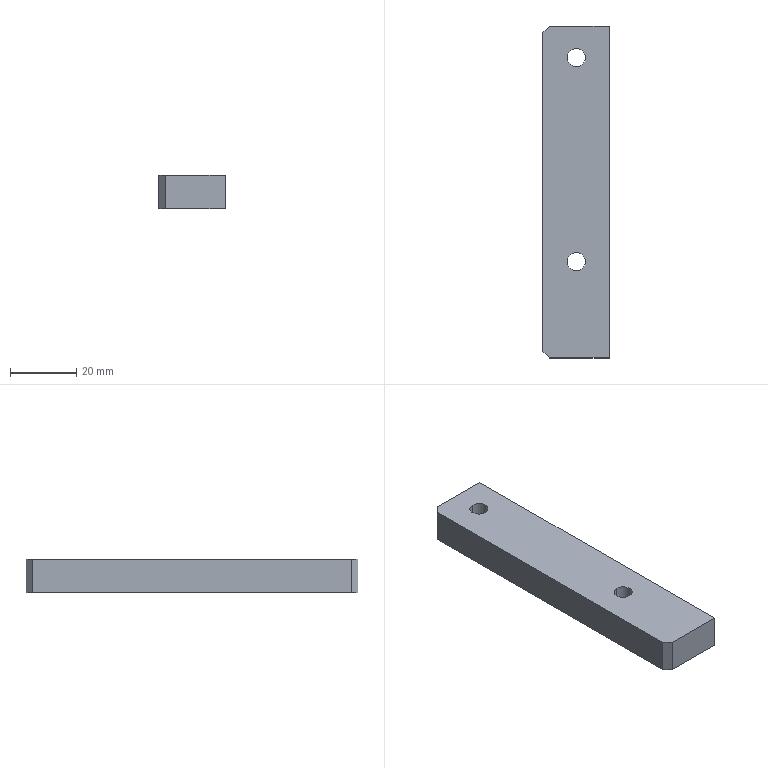Component | SolidWorks | BladeHolder-1 | 1 solid | 18 faces | box 20 x 100 x 10 mm | volume 18828 mm3 | plane 10 | cylinder 8 | commonest cylinder face diameters 12.238 x4 5.5 x4
build123d program:
from build123d import *

# Parameters (mm, degrees)
BOSS_EXTRUDE1_DEPTH                     = 10
M5_HEX_HEAD_BOLT_POST_HOLE1_D           = 5.5
M5_HEX_HEAD_BOLT_POST_HOLE1_CBORE_D     = 12.238
M5_HEX_HEAD_BOLT_POST_HOLE1_CBORE_DEPTH = 3.5


with BuildPart() as part:
    # Sketch1 → Boss-Extrude1 (new body)
    with BuildSketch(Plane.XY):
        Polygon((-48, 25), (-50, 23), (-50, 5), (50, 5), (50, 23), (48, 25), align=None)
    extrude(amount=BOSS_EXTRUDE1_DEPTH)

    # M5 Hex Head Bolt Post Hole1 (through all)
    with Locations(Plane.XY.offset(10)):
        with Locations((-40.5, 14.895), (21, 14.895)):
            CounterBoreHole(M5_HEX_HEAD_BOLT_POST_HOLE1_D / 2, M5_HEX_HEAD_BOLT_POST_HOLE1_CBORE_D / 2, M5_HEX_HEAD_BOLT_POST_HOLE1_CBORE_DEPTH)


solid = part.part

# Placed as in the assembly
solid = solid.moved(Location((-399.772, -298.766, 893.7), (180, 0, 90)))
STEP:
#1=COLOUR_RGB('',0.7922,0.8196,0.9333);
#2=FILL_AREA_STYLE_COLOUR('',#1);
#3=FILL_AREA_STYLE('',(#2));
#4=SURFACE_STYLE_FILL_AREA(#3);
#5=SURFACE_SIDE_STYLE('',(#4));
#6=SURFACE_STYLE_USAGE(.BOTH.,#5);
#7=PRESENTATION_STYLE_ASSIGNMENT((#6));
#8=CARTESIAN_POINT('',(-16.325,-9.927,34.929));
#9=VERTEX_POINT('',#8);
#10=CARTESIAN_POINT('',(-16.325,-10.409,34.929));
#11=VERTEX_POINT('',#10);
#12=CARTESIAN_POINT('',(-16.325,-10.168,34.929));
#13=DIRECTION('',(0.,0.,-1.));
#14=DIRECTION('',(0.,-1.,0.));
#15=AXIS2_PLACEMENT_3D('',#12,#13,#14);
#16=CIRCLE('',#15,0.2409);
#17=EDGE_CURVE('',#9,#11,#16,.T.);
#18=ORIENTED_EDGE('',*,*,#17,.F.);
#19=CARTESIAN_POINT('',(-16.325,-9.927,34.791));
#20=VERTEX_POINT('',#19);
#21=CARTESIAN_POINT('',(-16.325,-9.927,34.791));
#22=DIRECTION('',(0.,0.,-1.));
#23=VECTOR('',#22,39.37);
#24=LINE('',#21,#23);
#25=EDGE_CURVE('',#9,#20,#24,.T.);
#26=ORIENTED_EDGE('',*,*,#25,.T.);
#27=CARTESIAN_POINT('',(-16.325,-10.409,34.791));
#28=VERTEX_POINT('',#27);
#29=CARTESIAN_POINT('',(-16.325,-10.168,34.791));
#30=DIRECTION('',(0.,0.,-1.));
#31=DIRECTION('',(0.,-1.,0.));
#32=AXIS2_PLACEMENT_3D('',#29,#30,#31);
#33=CIRCLE('',#32,0.2409);
#34=EDGE_CURVE('',#20,#28,#33,.T.);
#35=ORIENTED_EDGE('',*,*,#34,.T.);
#36=CARTESIAN_POINT('',(-16.325,-10.409,34.791));
#37=DIRECTION('',(0.,0.,-1.));
#38=VECTOR('',#37,39.37);
#39=LINE('',#36,#38);
#40=EDGE_CURVE('',#11,#28,#39,.T.);
#41=ORIENTED_EDGE('',*,*,#40,.F.);
#42=EDGE_LOOP('',(#18,#26,#35,#41));
#43=FACE_OUTER_BOUND('',#42,.T.);
#44=CARTESIAN_POINT('',(-16.325,-10.168,34.791));
#45=DIRECTION('',(0.,0.,-1.));
#46=DIRECTION('',(0.,-1.,0.));
#47=AXIS2_PLACEMENT_3D('',#44,#45,#46);
#48=CYLINDRICAL_SURFACE('',#47,0.2409);
#49=ADVANCED_FACE('',(#43),#48,.F.);
#50=CARTESIAN_POINT('',(-16.325,-10.06,35.185));
#51=VERTEX_POINT('',#50);
#52=CARTESIAN_POINT('',(-16.325,-10.276,35.185));
#53=VERTEX_POINT('',#52);
#54=CARTESIAN_POINT('',(-16.325,-10.168,35.185));
#55=DIRECTION('',(0.,0.,-1.));
#56=DIRECTION('',(0.,-1.,0.));
#57=AXIS2_PLACEMENT_3D('',#54,#55,#56);
#58=CIRCLE('',#57,0.1083);
#59=EDGE_CURVE('',#51,#53,#58,.T.);
#60=ORIENTED_EDGE('',*,*,#59,.F.);
#61=CARTESIAN_POINT('',(-16.325,-10.06,34.929));
#62=VERTEX_POINT('',#61);
#63=CARTESIAN_POINT('',(-16.325,-10.06,34.791));
#64=DIRECTION('',(0.,0.,-1.));
#65=VECTOR('',#64,39.37);
#66=LINE('',#63,#65);
#67=EDGE_CURVE('',#51,#62,#66,.T.);
#68=ORIENTED_EDGE('',*,*,#67,.T.);
#69=CARTESIAN_POINT('',(-16.325,-10.276,34.929));
#70=VERTEX_POINT('',#69);
#71=CARTESIAN_POINT('',(-16.325,-10.168,34.929));
#72=DIRECTION('',(0.,0.,-1.));
#73=DIRECTION('',(0.,-1.,0.));
#74=AXIS2_PLACEMENT_3D('',#71,#72,#73);
#75=CIRCLE('',#74,0.1083);
#76=EDGE_CURVE('',#62,#70,#75,.T.);
#77=ORIENTED_EDGE('',*,*,#76,.T.);
#78=CARTESIAN_POINT('',(-16.325,-10.276,34.791));
#79=DIRECTION('',(0.,0.,-1.));
#80=VECTOR('',#79,39.37);
#81=LINE('',#78,#80);
#82=EDGE_CURVE('',#53,#70,#81,.T.);
#83=ORIENTED_EDGE('',*,*,#82,.F.);
#84=EDGE_LOOP('',(#60,#68,#77,#83));
#85=FACE_OUTER_BOUND('',#84,.T.);
#86=CARTESIAN_POINT('',(-16.325,-10.168,34.791));
#87=DIRECTION('',(0.,0.,-1.));
#88=DIRECTION('',(0.,-1.,0.));
#89=AXIS2_PLACEMENT_3D('',#86,#87,#88);
#90=CYLINDRICAL_SURFACE('',#89,0.1083);
#91=ADVANCED_FACE('',(#85),#90,.F.);
#92=CARTESIAN_POINT('',(-16.325,-12.348,34.929));
#93=VERTEX_POINT('',#92);
#94=CARTESIAN_POINT('',(-16.325,-12.83,34.929));
#95=VERTEX_POINT('',#94);
#96=CARTESIAN_POINT('',(-16.325,-12.589,34.929));
#97=DIRECTION('',(0.,0.,-1.));
#98=DIRECTION('',(0.,-1.,0.));
#99=AXIS2_PLACEMENT_3D('',#96,#97,#98);
#100=CIRCLE('',#99,0.2409);
#101=EDGE_CURVE('',#93,#95,#100,.T.);
#102=ORIENTED_EDGE('',*,*,#101,.F.);
#103=CARTESIAN_POINT('',(-16.325,-12.348,34.791));
#104=VERTEX_POINT('',#103);
#105=CARTESIAN_POINT('',(-16.325,-12.348,34.791));
#106=DIRECTION('',(0.,0.,-1.));
#107=VECTOR('',#106,39.37);
#108=LINE('',#105,#107);
#109=EDGE_CURVE('',#93,#104,#108,.T.);
#110=ORIENTED_EDGE('',*,*,#109,.T.);
#111=CARTESIAN_POINT('',(-16.325,-12.83,34.791));
#112=VERTEX_POINT('',#111);
#113=CARTESIAN_POINT('',(-16.325,-12.589,34.791));
#114=DIRECTION('',(0.,0.,-1.));
#115=DIRECTION('',(0.,-1.,0.));
#116=AXIS2_PLACEMENT_3D('',#113,#114,#115);
#117=CIRCLE('',#116,0.2409);
#118=EDGE_CURVE('',#104,#112,#117,.T.);
#119=ORIENTED_EDGE('',*,*,#118,.T.);
#120=CARTESIAN_POINT('',(-16.325,-12.83,34.791));
#121=DIRECTION('',(0.,0.,-1.));
#122=VECTOR('',#121,39.37);
#123=LINE('',#120,#122);
#124=EDGE_CURVE('',#95,#112,#123,.T.);
#125=ORIENTED_EDGE('',*,*,#124,.F.);
#126=EDGE_LOOP('',(#102,#110,#119,#125));
#127=FACE_OUTER_BOUND('',#126,.T.);
#128=CARTESIAN_POINT('',(-16.325,-12.589,34.791));
#129=DIRECTION('',(0.,0.,-1.));
#130=DIRECTION('',(0.,-1.,0.));
#131=AXIS2_PLACEMENT_3D('',#128,#129,#130);
#132=CYLINDRICAL_SURFACE('',#131,0.2409);
#133=ADVANCED_FACE('',(#127),#132,.F.);
#134=CARTESIAN_POINT('',(-16.325,-12.481,35.185));
#135=VERTEX_POINT('',#134);
#136=CARTESIAN_POINT('',(-16.325,-12.697,35.185));
#137=VERTEX_POINT('',#136);
#138=CARTESIAN_POINT('',(-16.325,-12.589,35.185));
#139=DIRECTION('',(0.,0.,-1.));
#140=DIRECTION('',(0.,-1.,0.));
#141=AXIS2_PLACEMENT_3D('',#138,#139,#140);
#142=CIRCLE('',#141,0.1083);
#143=EDGE_CURVE('',#135,#137,#142,.T.);
#144=ORIENTED_EDGE('',*,*,#143,.F.);
#145=CARTESIAN_POINT('',(-16.325,-12.481,34.929));
#146=VERTEX_POINT('',#145);
#147=CARTESIAN_POINT('',(-16.325,-12.481,34.791));
#148=DIRECTION('',(0.,0.,-1.));
#149=VECTOR('',#148,39.37);
#150=LINE('',#147,#149);
#151=EDGE_CURVE('',#135,#146,#150,.T.);
#152=ORIENTED_EDGE('',*,*,#151,.T.);
#153=CARTESIAN_POINT('',(-16.325,-12.697,34.929));
#154=VERTEX_POINT('',#153);
#155=CARTESIAN_POINT('',(-16.325,-12.589,34.929));
#156=DIRECTION('',(0.,0.,-1.));
#157=DIRECTION('',(0.,-1.,0.));
#158=AXIS2_PLACEMENT_3D('',#155,#156,#157);
#159=CIRCLE('',#158,0.1083);
#160=EDGE_CURVE('',#146,#154,#159,.T.);
#161=ORIENTED_EDGE('',*,*,#160,.T.);
#162=CARTESIAN_POINT('',(-16.325,-12.697,34.791));
#163=DIRECTION('',(0.,0.,-1.));
#164=VECTOR('',#163,39.37);
#165=LINE('',#162,#164);
#166=EDGE_CURVE('',#137,#154,#165,.T.);
#167=ORIENTED_EDGE('',*,*,#166,.F.);
#168=EDGE_LOOP('',(#144,#152,#161,#167));
#169=FACE_OUTER_BOUND('',#168,.T.);
#170=CARTESIAN_POINT('',(-16.325,-12.589,34.791));
#171=DIRECTION('',(0.,0.,-1.));
#172=DIRECTION('',(0.,-1.,0.));
#173=AXIS2_PLACEMENT_3D('',#170,#171,#172);
#174=CYLINDRICAL_SURFACE('',#173,0.1083);
#175=ADVANCED_FACE('',(#169),#174,.F.);
#176=CARTESIAN_POINT('',(-15.936,-13.731,35.185));
#177=VERTEX_POINT('',#176);
#178=CARTESIAN_POINT('',(-16.645,-13.731,35.185));
#179=VERTEX_POINT('',#178);
#180=CARTESIAN_POINT('',(-16.645,-13.731,35.185));
#181=DIRECTION('',(-1.,-0.,-0.));
#182=VECTOR('',#181,39.37);
#183=LINE('',#180,#182);
#184=EDGE_CURVE('',#177,#179,#183,.T.);
#185=ORIENTED_EDGE('',*,*,#184,.T.);
#186=CARTESIAN_POINT('',(-16.645,-13.731,34.791));
#187=VERTEX_POINT('',#186);
#188=CARTESIAN_POINT('',(-16.645,-13.731,34.791));
#189=DIRECTION('',(-0.,-0.,1.));
#190=VECTOR('',#189,39.37);
#191=LINE('',#188,#190);
#192=EDGE_CURVE('',#187,#179,#191,.T.);
#193=ORIENTED_EDGE('',*,*,#192,.F.);
#194=CARTESIAN_POINT('',(-15.936,-13.731,34.791));
#195=VERTEX_POINT('',#194);
#196=CARTESIAN_POINT('',(-16.645,-13.731,34.791));
#197=DIRECTION('',(-1.,-0.,-0.));
#198=VECTOR('',#197,39.37);
#199=LINE('',#196,#198);
#200=EDGE_CURVE('',#195,#187,#199,.T.);
#201=ORIENTED_EDGE('',*,*,#200,.F.);
#202=CARTESIAN_POINT('',(-15.936,-13.731,34.791));
#203=DIRECTION('',(-0.,-0.,1.));
#204=VECTOR('',#203,39.37);
#205=LINE('',#202,#204);
#206=EDGE_CURVE('',#195,#177,#205,.T.);
#207=ORIENTED_EDGE('',*,*,#206,.T.);
#208=EDGE_LOOP('',(#185,#193,#201,#207));
#209=FACE_OUTER_BOUND('',#208,.T.);
#210=CARTESIAN_POINT('',(-16.645,-13.731,34.791));
#211=DIRECTION('',(-0.,1.,0.));
#212=DIRECTION('',(0.,0.,-1.));
#213=AXIS2_PLACEMENT_3D('',#210,#211,#212);
#214=PLANE('',#213);
#215=ADVANCED_FACE('',(#209),#214,.F.);
#216=CARTESIAN_POINT('',(-16.723,-13.652,35.185));
#217=VERTEX_POINT('',#216);
#218=CARTESIAN_POINT('',(-16.723,-13.652,35.185));
#219=DIRECTION('',(-0.7071,0.7071,0.));
#220=VECTOR('',#219,39.37);
#221=LINE('',#218,#220);
#222=EDGE_CURVE('',#179,#217,#221,.T.);
#223=ORIENTED_EDGE('',*,*,#222,.T.);
#224=CARTESIAN_POINT('',(-16.723,-13.652,34.791));
#225=VERTEX_POINT('',#224);
#226=CARTESIAN_POINT('',(-16.723,-13.652,34.791));
#227=DIRECTION('',(-0.,-0.,1.));
#228=VECTOR('',#227,39.37);
#229=LINE('',#226,#228);
#230=EDGE_CURVE('',#225,#217,#229,.T.);
#231=ORIENTED_EDGE('',*,*,#230,.F.);
#232=CARTESIAN_POINT('',(-16.723,-13.652,34.791));
#233=DIRECTION('',(-0.7071,0.7071,0.));
#234=VECTOR('',#233,39.37);
#235=LINE('',#232,#234);
#236=EDGE_CURVE('',#187,#225,#235,.T.);
#237=ORIENTED_EDGE('',*,*,#236,.F.);
#238=ORIENTED_EDGE('',*,*,#192,.T.);
#239=EDGE_LOOP('',(#223,#231,#237,#238));
#240=FACE_OUTER_BOUND('',#239,.T.);
#241=CARTESIAN_POINT('',(-16.723,-13.652,34.791));
#242=DIRECTION('',(0.7071,0.7071,0.));
#243=DIRECTION('',(0.7071,-0.7071,-0.));
#244=AXIS2_PLACEMENT_3D('',#241,#242,#243);
#245=PLANE('',#244);
#246=ADVANCED_FACE('',(#240),#245,.F.);
#247=CARTESIAN_POINT('',(-16.723,-9.873,35.185));
#248=VERTEX_POINT('',#247);
#249=CARTESIAN_POINT('',(-16.723,-9.873,35.185));
#250=DIRECTION('',(-0.,1.,0.));
#251=VECTOR('',#250,39.37);
#252=LINE('',#249,#251);
#253=EDGE_CURVE('',#217,#248,#252,.T.);
#254=ORIENTED_EDGE('',*,*,#253,.T.);
#255=CARTESIAN_POINT('',(-16.723,-9.873,34.791));
#256=VERTEX_POINT('',#255);
#257=CARTESIAN_POINT('',(-16.723,-9.873,34.791));
#258=DIRECTION('',(-0.,-0.,1.));
#259=VECTOR('',#258,39.37);
#260=LINE('',#257,#259);
#261=EDGE_CURVE('',#256,#248,#260,.T.);
#262=ORIENTED_EDGE('',*,*,#261,.F.);
#263=CARTESIAN_POINT('',(-16.723,-9.873,34.791));
#264=DIRECTION('',(-0.,1.,0.));
#265=VECTOR('',#264,39.37);
#266=LINE('',#263,#265);
#267=EDGE_CURVE('',#225,#256,#266,.T.);
#268=ORIENTED_EDGE('',*,*,#267,.F.);
#269=ORIENTED_EDGE('',*,*,#230,.T.);
#270=EDGE_LOOP('',(#254,#262,#268,#269));
#271=FACE_OUTER_BOUND('',#270,.T.);
#272=CARTESIAN_POINT('',(-16.723,-9.873,34.791));
#273=DIRECTION('',(1.,0.,0.));
#274=DIRECTION('',(-0.,-0.,1.));
#275=AXIS2_PLACEMENT_3D('',#272,#273,#274);
#276=PLANE('',#275);
#277=ADVANCED_FACE('',(#271),#276,.F.);
#278=CARTESIAN_POINT('',(-16.645,-9.794,35.185));
#279=VERTEX_POINT('',#278);
#280=CARTESIAN_POINT('',(-16.723,-9.873,35.185));
#281=DIRECTION('',(0.7071,0.7071,0.));
#282=VECTOR('',#281,39.37);
#283=LINE('',#280,#282);
#284=EDGE_CURVE('',#248,#279,#283,.T.);
#285=ORIENTED_EDGE('',*,*,#284,.T.);
#286=CARTESIAN_POINT('',(-16.645,-9.794,34.791));
#287=VERTEX_POINT('',#286);
#288=CARTESIAN_POINT('',(-16.645,-9.794,34.791));
#289=DIRECTION('',(-0.,-0.,1.));
#290=VECTOR('',#289,39.37);
#291=LINE('',#288,#290);
#292=EDGE_CURVE('',#287,#279,#291,.T.);
#293=ORIENTED_EDGE('',*,*,#292,.F.);
#294=CARTESIAN_POINT('',(-16.723,-9.873,34.791));
#295=DIRECTION('',(0.7071,0.7071,0.));
#296=VECTOR('',#295,39.37);
#297=LINE('',#294,#296);
#298=EDGE_CURVE('',#256,#287,#297,.T.);
#299=ORIENTED_EDGE('',*,*,#298,.F.);
#300=ORIENTED_EDGE('',*,*,#261,.T.);
#301=EDGE_LOOP('',(#285,#293,#299,#300));
#302=FACE_OUTER_BOUND('',#301,.T.);
#303=CARTESIAN_POINT('',(-16.723,-9.873,34.791));
#304=DIRECTION('',(0.7071,-0.7071,-0.));
#305=DIRECTION('',(-0.7071,-0.7071,-0.));
#306=AXIS2_PLACEMENT_3D('',#303,#304,#305);
#307=PLANE('',#306);
#308=ADVANCED_FACE('',(#302),#307,.F.);
#309=CARTESIAN_POINT('',(-15.936,-9.794,35.185));
#310=VERTEX_POINT('',#309);
#311=CARTESIAN_POINT('',(-16.645,-9.794,35.185));
#312=DIRECTION('',(1.,0.,0.));
#313=VECTOR('',#312,39.37);
#314=LINE('',#311,#313);
#315=EDGE_CURVE('',#279,#310,#314,.T.);
#316=ORIENTED_EDGE('',*,*,#315,.T.);
#317=CARTESIAN_POINT('',(-15.936,-9.794,34.791));
#318=VERTEX_POINT('',#317);
#319=CARTESIAN_POINT('',(-15.936,-9.794,34.791));
#320=DIRECTION('',(-0.,-0.,1.));
#321=VECTOR('',#320,39.37);
#322=LINE('',#319,#321);
#323=EDGE_CURVE('',#318,#310,#322,.T.);
#324=ORIENTED_EDGE('',*,*,#323,.F.);
#325=CARTESIAN_POINT('',(-16.645,-9.794,34.791));
#326=DIRECTION('',(1.,0.,0.));
#327=VECTOR('',#326,39.37);
#328=LINE('',#325,#327);
#329=EDGE_CURVE('',#287,#318,#328,.T.);
#330=ORIENTED_EDGE('',*,*,#329,.F.);
#331=ORIENTED_EDGE('',*,*,#292,.T.);
#332=EDGE_LOOP('',(#316,#324,#330,#331));
#333=FACE_OUTER_BOUND('',#332,.T.);
#334=CARTESIAN_POINT('',(-16.645,-9.794,34.791));
#335=DIRECTION('',(0.,-1.,-0.));
#336=DIRECTION('',(-0.,-0.,1.));
#337=AXIS2_PLACEMENT_3D('',#334,#335,#336);
#338=PLANE('',#337);
#339=ADVANCED_FACE('',(#333),#338,.F.);
#340=CARTESIAN_POINT('',(-15.936,-9.794,35.185));
#341=DIRECTION('',(0.,-1.,-0.));
#342=VECTOR('',#341,39.37);
#343=LINE('',#340,#342);
#344=EDGE_CURVE('',#310,#177,#343,.T.);
#345=ORIENTED_EDGE('',*,*,#344,.T.);
#346=ORIENTED_EDGE('',*,*,#206,.F.);
#347=CARTESIAN_POINT('',(-15.936,-9.794,34.791));
#348=DIRECTION('',(0.,-1.,-0.));
#349=VECTOR('',#348,39.37);
#350=LINE('',#347,#349);
#351=EDGE_CURVE('',#318,#195,#350,.T.);
#352=ORIENTED_EDGE('',*,*,#351,.F.);
#353=ORIENTED_EDGE('',*,*,#323,.T.);
#354=EDGE_LOOP('',(#345,#346,#352,#353));
#355=FACE_OUTER_BOUND('',#354,.T.);
#356=CARTESIAN_POINT('',(-15.936,-9.794,34.791));
#357=DIRECTION('',(-1.,-0.,-0.));
#358=DIRECTION('',(0.,0.,-1.));
#359=AXIS2_PLACEMENT_3D('',#356,#357,#358);
#360=PLANE('',#359);
#361=ADVANCED_FACE('',(#355),#360,.F.);
#362=CARTESIAN_POINT('',(-16.325,-10.168,34.791));
#363=DIRECTION('',(0.,0.,-1.));
#364=DIRECTION('',(0.,-1.,0.));
#365=AXIS2_PLACEMENT_3D('',#362,#363,#364);
#366=CIRCLE('',#365,0.2409);
#367=EDGE_CURVE('',#28,#20,#366,.T.);
#368=ORIENTED_EDGE('',*,*,#367,.F.);
#369=ORIENTED_EDGE('',*,*,#34,.F.);
#370=EDGE_LOOP('',(#368,#369));
#371=FACE_BOUND('',#370,.T.);
#372=CARTESIAN_POINT('',(-16.325,-12.589,34.791));
#373=DIRECTION('',(0.,0.,-1.));
#374=DIRECTION('',(0.,-1.,0.));
#375=AXIS2_PLACEMENT_3D('',#372,#373,#374);
#376=CIRCLE('',#375,0.2409);
#377=EDGE_CURVE('',#112,#104,#376,.T.);
#378=ORIENTED_EDGE('',*,*,#377,.F.);
#379=ORIENTED_EDGE('',*,*,#118,.F.);
#380=EDGE_LOOP('',(#378,#379));
#381=FACE_BOUND('',#380,.T.);
#382=ORIENTED_EDGE('',*,*,#200,.T.);
#383=ORIENTED_EDGE('',*,*,#236,.T.);
#384=ORIENTED_EDGE('',*,*,#267,.T.);
#385=ORIENTED_EDGE('',*,*,#298,.T.);
#386=ORIENTED_EDGE('',*,*,#329,.T.);
#387=ORIENTED_EDGE('',*,*,#351,.T.);
#388=EDGE_LOOP('',(#382,#383,#384,#385,#386,#387));
#389=FACE_OUTER_BOUND('',#388,.T.);
#390=CARTESIAN_POINT('',(-15.739,-11.762,34.791));
#391=DIRECTION('',(0.,0.,-1.));
#392=DIRECTION('',(0.,-1.,-0.));
#393=AXIS2_PLACEMENT_3D('',#390,#391,#392);
#394=PLANE('',#393);
#395=ADVANCED_FACE('',(#371,#381,#389),#394,.T.);
#396=CARTESIAN_POINT('',(-16.325,-10.168,35.185));
#397=DIRECTION('',(0.,0.,-1.));
#398=DIRECTION('',(0.,-1.,0.));
#399=AXIS2_PLACEMENT_3D('',#396,#397,#398);
#400=CIRCLE('',#399,0.1083);
#401=EDGE_CURVE('',#53,#51,#400,.T.);
#402=ORIENTED_EDGE('',*,*,#401,.T.);
#403=ORIENTED_EDGE('',*,*,#59,.T.);
#404=EDGE_LOOP('',(#402,#403));
#405=FACE_BOUND('',#404,.T.);
#406=CARTESIAN_POINT('',(-16.325,-12.589,35.185));
#407=DIRECTION('',(0.,0.,-1.));
#408=DIRECTION('',(0.,-1.,0.));
#409=AXIS2_PLACEMENT_3D('',#406,#407,#408);
#410=CIRCLE('',#409,0.1083);
#411=EDGE_CURVE('',#137,#135,#410,.T.);
#412=ORIENTED_EDGE('',*,*,#411,.T.);
#413=ORIENTED_EDGE('',*,*,#143,.T.);
#414=EDGE_LOOP('',(#412,#413));
#415=FACE_BOUND('',#414,.T.);
#416=ORIENTED_EDGE('',*,*,#184,.F.);
#417=ORIENTED_EDGE('',*,*,#344,.F.);
#418=ORIENTED_EDGE('',*,*,#315,.F.);
#419=ORIENTED_EDGE('',*,*,#284,.F.);
#420=ORIENTED_EDGE('',*,*,#253,.F.);
#421=ORIENTED_EDGE('',*,*,#222,.F.);
#422=EDGE_LOOP('',(#416,#417,#418,#419,#420,#421));
#423=FACE_OUTER_BOUND('',#422,.T.);
#424=CARTESIAN_POINT('',(-15.739,-11.762,35.185));
#425=DIRECTION('',(0.,0.,-1.));
#426=DIRECTION('',(0.,-1.,-0.));
#427=AXIS2_PLACEMENT_3D('',#424,#425,#426);
#428=PLANE('',#427);
#429=ADVANCED_FACE('',(#405,#415,#423),#428,.F.);
#430=ORIENTED_EDGE('',*,*,#151,.F.);
#431=ORIENTED_EDGE('',*,*,#411,.F.);
#432=ORIENTED_EDGE('',*,*,#166,.T.);
#433=CARTESIAN_POINT('',(-16.325,-12.589,34.929));
#434=DIRECTION('',(0.,0.,-1.));
#435=DIRECTION('',(0.,-1.,0.));
#436=AXIS2_PLACEMENT_3D('',#433,#434,#435);
#437=CIRCLE('',#436,0.1083);
#438=EDGE_CURVE('',#154,#146,#437,.T.);
#439=ORIENTED_EDGE('',*,*,#438,.T.);
#440=EDGE_LOOP('',(#430,#431,#432,#439));
#441=FACE_OUTER_BOUND('',#440,.T.);
#442=CARTESIAN_POINT('',(-16.325,-12.589,34.791));
#443=DIRECTION('',(0.,0.,-1.));
#444=DIRECTION('',(0.,-1.,0.));
#445=AXIS2_PLACEMENT_3D('',#442,#443,#444);
#446=CYLINDRICAL_SURFACE('',#445,0.1083);
#447=ADVANCED_FACE('',(#441),#446,.F.);
#448=ORIENTED_EDGE('',*,*,#438,.F.);
#449=ORIENTED_EDGE('',*,*,#160,.F.);
#450=EDGE_LOOP('',(#448,#449));
#451=FACE_BOUND('',#450,.T.);
#452=CARTESIAN_POINT('',(-16.325,-12.589,34.929));
#453=DIRECTION('',(0.,0.,-1.));
#454=DIRECTION('',(0.,-1.,0.));
#455=AXIS2_PLACEMENT_3D('',#452,#453,#454);
#456=CIRCLE('',#455,0.2409);
#457=EDGE_CURVE('',#95,#93,#456,.T.);
#458=ORIENTED_EDGE('',*,*,#457,.T.);
#459=ORIENTED_EDGE('',*,*,#101,.T.);
#460=EDGE_LOOP('',(#458,#459));
#461=FACE_OUTER_BOUND('',#460,.T.);
#462=CARTESIAN_POINT('',(-16.325,-12.697,34.929));
#463=DIRECTION('',(-0.,-0.,1.));
#464=DIRECTION('',(-0.,1.,0.));
#465=AXIS2_PLACEMENT_3D('',#462,#463,#464);
#466=PLANE('',#465);
#467=ADVANCED_FACE('',(#451,#461),#466,.F.);
#468=ORIENTED_EDGE('',*,*,#109,.F.);
#469=ORIENTED_EDGE('',*,*,#457,.F.);
#470=ORIENTED_EDGE('',*,*,#124,.T.);
#471=ORIENTED_EDGE('',*,*,#377,.T.);
#472=EDGE_LOOP('',(#468,#469,#470,#471));
#473=FACE_OUTER_BOUND('',#472,.T.);
#474=CARTESIAN_POINT('',(-16.325,-12.589,34.791));
#475=DIRECTION('',(0.,0.,-1.));
#476=DIRECTION('',(0.,-1.,0.));
#477=AXIS2_PLACEMENT_3D('',#474,#475,#476);
#478=CYLINDRICAL_SURFACE('',#477,0.2409);
#479=ADVANCED_FACE('',(#473),#478,.F.);
#480=ORIENTED_EDGE('',*,*,#67,.F.);
#481=ORIENTED_EDGE('',*,*,#401,.F.);
#482=ORIENTED_EDGE('',*,*,#82,.T.);
#483=CARTESIAN_POINT('',(-16.325,-10.168,34.929));
#484=DIRECTION('',(0.,0.,-1.));
#485=DIRECTION('',(0.,-1.,0.));
#486=AXIS2_PLACEMENT_3D('',#483,#484,#485);
#487=CIRCLE('',#486,0.1083);
#488=EDGE_CURVE('',#70,#62,#487,.T.);
#489=ORIENTED_EDGE('',*,*,#488,.T.);
#490=EDGE_LOOP('',(#480,#481,#482,#489));
#491=FACE_OUTER_BOUND('',#490,.T.);
#492=CARTESIAN_POINT('',(-16.325,-10.168,34.791));
#493=DIRECTION('',(0.,0.,-1.));
#494=DIRECTION('',(0.,-1.,0.));
#495=AXIS2_PLACEMENT_3D('',#492,#493,#494);
#496=CYLINDRICAL_SURFACE('',#495,0.1083);
#497=ADVANCED_FACE('',(#491),#496,.F.);
#498=ORIENTED_EDGE('',*,*,#488,.F.);
#499=ORIENTED_EDGE('',*,*,#76,.F.);
#500=EDGE_LOOP('',(#498,#499));
#501=FACE_BOUND('',#500,.T.);
#502=CARTESIAN_POINT('',(-16.325,-10.168,34.929));
#503=DIRECTION('',(0.,0.,-1.));
#504=DIRECTION('',(0.,-1.,0.));
#505=AXIS2_PLACEMENT_3D('',#502,#503,#504);
#506=CIRCLE('',#505,0.2409);
#507=EDGE_CURVE('',#11,#9,#506,.T.);
#508=ORIENTED_EDGE('',*,*,#507,.T.);
#509=ORIENTED_EDGE('',*,*,#17,.T.);
#510=EDGE_LOOP('',(#508,#509));
#511=FACE_OUTER_BOUND('',#510,.T.);
#512=CARTESIAN_POINT('',(-16.325,-10.276,34.929));
#513=DIRECTION('',(-0.,-0.,1.));
#514=DIRECTION('',(-0.,1.,0.));
#515=AXIS2_PLACEMENT_3D('',#512,#513,#514);
#516=PLANE('',#515);
#517=ADVANCED_FACE('',(#501,#511),#516,.F.);
#518=ORIENTED_EDGE('',*,*,#25,.F.);
#519=ORIENTED_EDGE('',*,*,#507,.F.);
#520=ORIENTED_EDGE('',*,*,#40,.T.);
#521=ORIENTED_EDGE('',*,*,#367,.T.);
#522=EDGE_LOOP('',(#518,#519,#520,#521));
#523=FACE_OUTER_BOUND('',#522,.T.);
#524=CARTESIAN_POINT('',(-16.325,-10.168,34.791));
#525=DIRECTION('',(0.,0.,-1.));
#526=DIRECTION('',(0.,-1.,0.));
#527=AXIS2_PLACEMENT_3D('',#524,#525,#526);
#528=CYLINDRICAL_SURFACE('',#527,0.2409);
#529=ADVANCED_FACE('',(#523),#528,.F.);
#530=CLOSED_SHELL('',(#49,#91,#133,#175,#215,#246,#277,#308,#339,#361,#395,#429,#447,#467,#479,#497,#517,#529));
#531=MANIFOLD_SOLID_BREP('',#530);
#532=STYLED_ITEM('',(#7),#531);
#533=(LENGTH_UNIT()NAMED_UNIT(*)SI_UNIT($,.METRE.));
#534=LENGTH_MEASURE_WITH_UNIT(LENGTH_MEASURE(0.0254),#533);
#535=DIMENSIONAL_EXPONENTS(1.,0.,0.,0.,0.,0.,0.);
#536=(CONVERSION_BASED_UNIT('',#534)LENGTH_UNIT()NAMED_UNIT(#535));
#537=UNCERTAINTY_MEASURE_WITH_UNIT(LENGTH_MEASURE(0.00001),#536,'','');
#538=(NAMED_UNIT(*)PLANE_ANGLE_UNIT()SI_UNIT($,.RADIAN.));
#539=(NAMED_UNIT(*)SI_UNIT($,.STERADIAN.)SOLID_ANGLE_UNIT());
#540=(GEOMETRIC_REPRESENTATION_CONTEXT(3)GLOBAL_UNCERTAINTY_ASSIGNED_CONTEXT((#537))GLOBAL_UNIT_ASSIGNED_CONTEXT((#536,#538,#539))REPRESENTATION_CONTEXT('',''));
#541=MECHANICAL_DESIGN_GEOMETRIC_PRESENTATION_REPRESENTATION('',(#532),#540);
#542=CARTESIAN_POINT('',(0.,0.,0.));
#543=DIRECTION('',(0.,0.,1.));
#544=DIRECTION('',(1.,0.,0.));
#545=AXIS2_PLACEMENT_3D('',#542,#543,#544);
#546=(LENGTH_UNIT()NAMED_UNIT(*)SI_UNIT($,.METRE.));
#547=LENGTH_MEASURE_WITH_UNIT(LENGTH_MEASURE(0.0254),#546);
#548=DIMENSIONAL_EXPONENTS(1.,0.,0.,0.,0.,0.,0.);
#549=(CONVERSION_BASED_UNIT('',#547)LENGTH_UNIT()NAMED_UNIT(#548));
#550=UNCERTAINTY_MEASURE_WITH_UNIT(LENGTH_MEASURE(0.00001),#549,'','');
#551=(NAMED_UNIT(*)PLANE_ANGLE_UNIT()SI_UNIT($,.RADIAN.));
#552=(NAMED_UNIT(*)SI_UNIT($,.STERADIAN.)SOLID_ANGLE_UNIT());
#553=(GEOMETRIC_REPRESENTATION_CONTEXT(3)GLOBAL_UNCERTAINTY_ASSIGNED_CONTEXT((#550))GLOBAL_UNIT_ASSIGNED_CONTEXT((#549,#551,#552))REPRESENTATION_CONTEXT('',''));
#554=ADVANCED_BREP_SHAPE_REPRESENTATION('',(#531,#545),#553);
#555=PRESENTATION_LAYER_ASSIGNMENT('','',(#532));